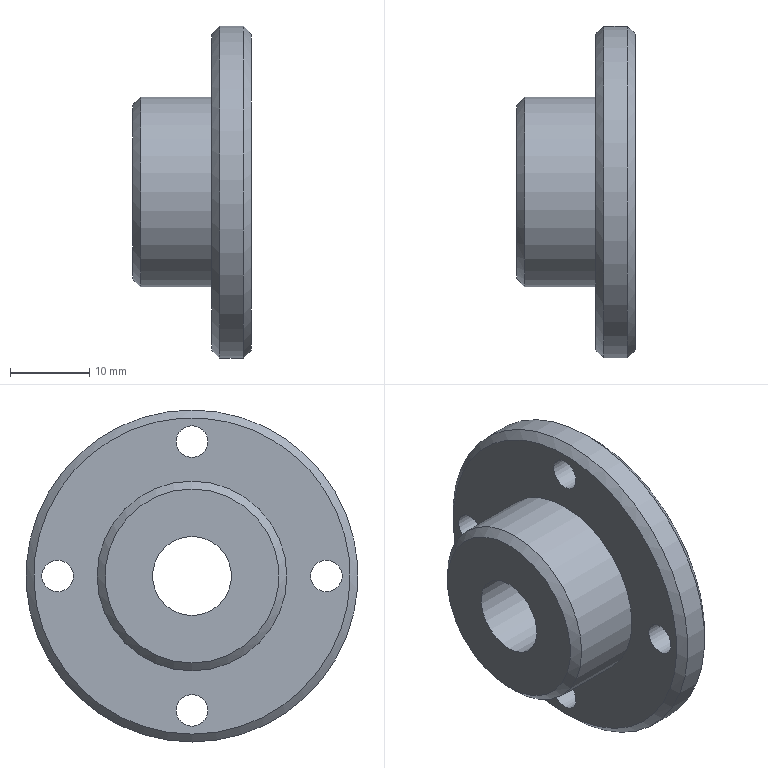Component | NX | CLAMP_PLATE | 1 solid | 16 faces | volume 9461 mm3 | cylinder 8 | plane 4 | cone 4 | commonest cylinder face diameters 4 x4 24 x1 42 x1 16 x1 10 x1